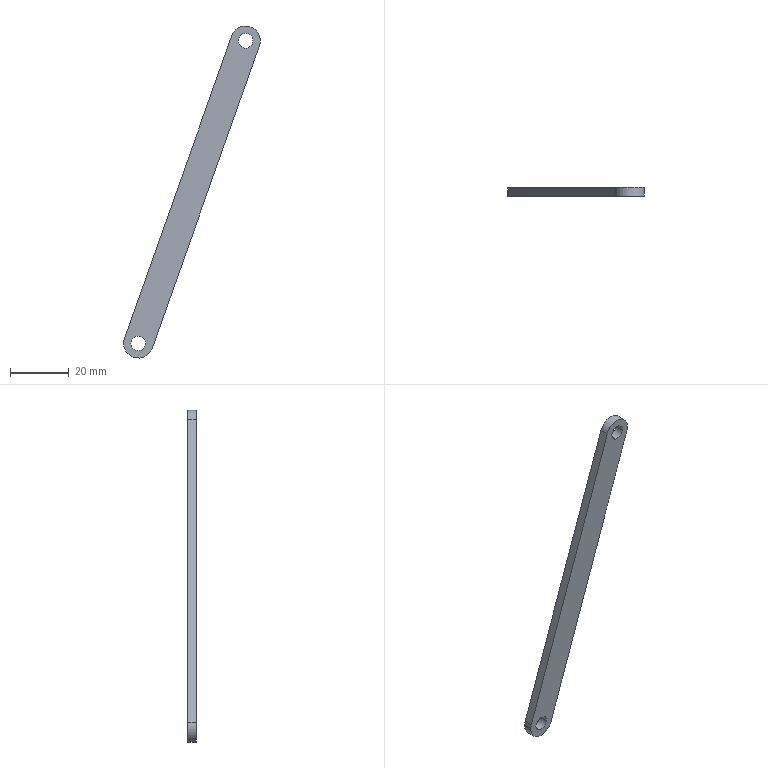Component | SolidWorks | WheelAssembly2-1_ConnectingRod2-1 | 1 solid | 11 faces | box 46.42 x 3 x 112.74 mm | volume 3388 mm3 | cylinder 7 | plane 4 | commonest cylinder face diameters 5 x4 10 x3
build123d program:
from build123d import *

# Parameters (mm, degrees)
SKETCH1_R           = 2.5
BOSS_EXTRUDE1_DEPTH = 3


with BuildPart() as part:
    # Sketch1 → Boss-Extrude1 (new body)
    with BuildSketch(Plane.XY):
        with BuildLine():
            Line((-54.5, 5), (54.5, 5))
            ThreePointArc((54.5, 5), (59.5, 0), (54.5, -5))
            Line((54.5, -5), (-54.5, -5))
            ThreePointArc((-54.5, -5), (-59.5, 0), (-54.5, 5))
        make_face()
        with Locations((-54.5, 0)):
            Circle(SKETCH1_R, mode=Mode.SUBTRACT)
        with Locations((54.5, 0)):
            Circle(SKETCH1_R, mode=Mode.SUBTRACT)
    extrude(amount=BOSS_EXTRUDE1_DEPTH)


solid = part.part

# Placed as in the assembly
solid = solid.moved(Location((-286.791, -33, -380.602), (-90, 0, -70.481)))
STEP:
#1=CARTESIAN_POINT('',(-10.607,-1.299,-13.055));
#2=VERTEX_POINT('',#1);
#3=CARTESIAN_POINT('',(-10.541,-1.299,-12.869));
#4=VERTEX_POINT('',#3);
#5=CARTESIAN_POINT('',(-10.574,-1.299,-12.962));
#6=DIRECTION('',(0.,-1.,0.));
#7=DIRECTION('',(0.3341,0.,0.9425));
#8=AXIS2_PLACEMENT_3D('',#5,#6,#7);
#9=CIRCLE('',#8,0.09843);
#10=EDGE_CURVE('',#2,#4,#9,.T.);
#11=ORIENTED_EDGE('',*,*,#10,.T.);
#12=CARTESIAN_POINT('',(-10.541,-1.181,-12.869));
#13=VERTEX_POINT('',#12);
#14=CARTESIAN_POINT('',(-10.541,-1.299,-12.869));
#15=DIRECTION('',(-0.,1.,-0.));
#16=VECTOR('',#15,39.37);
#17=LINE('',#14,#16);
#18=EDGE_CURVE('',#4,#13,#17,.T.);
#19=ORIENTED_EDGE('',*,*,#18,.T.);
#20=CARTESIAN_POINT('',(-10.607,-1.181,-13.055));
#21=VERTEX_POINT('',#20);
#22=CARTESIAN_POINT('',(-10.574,-1.181,-12.962));
#23=DIRECTION('',(0.,-1.,0.));
#24=DIRECTION('',(0.3341,0.,0.9425));
#25=AXIS2_PLACEMENT_3D('',#22,#23,#24);
#26=CIRCLE('',#25,0.09843);
#27=EDGE_CURVE('',#21,#13,#26,.T.);
#28=ORIENTED_EDGE('',*,*,#27,.F.);
#29=CARTESIAN_POINT('',(-10.607,-1.299,-13.055));
#30=DIRECTION('',(-0.,1.,-0.));
#31=VECTOR('',#30,39.37);
#32=LINE('',#29,#31);
#33=EDGE_CURVE('',#2,#21,#32,.T.);
#34=ORIENTED_EDGE('',*,*,#33,.F.);
#35=EDGE_LOOP('',(#11,#19,#28,#34));
#36=FACE_OUTER_BOUND('',#35,.T.);
#37=CARTESIAN_POINT('',(-10.574,-1.299,-12.962));
#38=DIRECTION('',(-0.,1.,-0.));
#39=DIRECTION('',(-0.3341,-0.,-0.9425));
#40=AXIS2_PLACEMENT_3D('',#37,#38,#39);
#41=CYLINDRICAL_SURFACE('',#40,0.09843);
#42=ADVANCED_FACE('',(#36),#41,.F.);
#43=CARTESIAN_POINT('',(-12.041,-1.299,-17.099));
#44=VERTEX_POINT('',#43);
#45=CARTESIAN_POINT('',(-11.975,-1.299,-16.914));
#46=VERTEX_POINT('',#45);
#47=CARTESIAN_POINT('',(-12.008,-1.299,-17.007));
#48=DIRECTION('',(0.,-1.,0.));
#49=DIRECTION('',(0.3341,0.,0.9425));
#50=AXIS2_PLACEMENT_3D('',#47,#48,#49);
#51=CIRCLE('',#50,0.09843);
#52=EDGE_CURVE('',#44,#46,#51,.T.);
#53=ORIENTED_EDGE('',*,*,#52,.T.);
#54=CARTESIAN_POINT('',(-11.975,-1.181,-16.914));
#55=VERTEX_POINT('',#54);
#56=CARTESIAN_POINT('',(-11.975,-1.299,-16.914));
#57=DIRECTION('',(-0.,1.,-0.));
#58=VECTOR('',#57,39.37);
#59=LINE('',#56,#58);
#60=EDGE_CURVE('',#46,#55,#59,.T.);
#61=ORIENTED_EDGE('',*,*,#60,.T.);
#62=CARTESIAN_POINT('',(-12.041,-1.181,-17.099));
#63=VERTEX_POINT('',#62);
#64=CARTESIAN_POINT('',(-12.008,-1.181,-17.007));
#65=DIRECTION('',(0.,-1.,0.));
#66=DIRECTION('',(0.3341,0.,0.9425));
#67=AXIS2_PLACEMENT_3D('',#64,#65,#66);
#68=CIRCLE('',#67,0.09843);
#69=EDGE_CURVE('',#63,#55,#68,.T.);
#70=ORIENTED_EDGE('',*,*,#69,.F.);
#71=CARTESIAN_POINT('',(-12.041,-1.299,-17.099));
#72=DIRECTION('',(-0.,1.,-0.));
#73=VECTOR('',#72,39.37);
#74=LINE('',#71,#73);
#75=EDGE_CURVE('',#44,#63,#74,.T.);
#76=ORIENTED_EDGE('',*,*,#75,.F.);
#77=EDGE_LOOP('',(#53,#61,#70,#76));
#78=FACE_OUTER_BOUND('',#77,.T.);
#79=CARTESIAN_POINT('',(-12.008,-1.299,-17.007));
#80=DIRECTION('',(-0.,1.,-0.));
#81=DIRECTION('',(-0.3341,-0.,-0.9425));
#82=AXIS2_PLACEMENT_3D('',#79,#80,#81);
#83=CYLINDRICAL_SURFACE('',#82,0.09843);
#84=ADVANCED_FACE('',(#78),#83,.F.);
#85=CARTESIAN_POINT('',(-12.074,-1.299,-17.192));
#86=VERTEX_POINT('',#85);
#87=CARTESIAN_POINT('',(-11.822,-1.299,-17.072));
#88=VERTEX_POINT('',#87);
#89=CARTESIAN_POINT('',(-12.008,-1.299,-17.007));
#90=DIRECTION('',(0.,-1.,0.));
#91=DIRECTION('',(0.3341,0.,0.9425));
#92=AXIS2_PLACEMENT_3D('',#89,#90,#91);
#93=CIRCLE('',#92,0.1969);
#94=EDGE_CURVE('',#86,#88,#93,.T.);
#95=ORIENTED_EDGE('',*,*,#94,.F.);
#96=CARTESIAN_POINT('',(-12.074,-1.181,-17.192));
#97=VERTEX_POINT('',#96);
#98=CARTESIAN_POINT('',(-12.074,-1.299,-17.192));
#99=DIRECTION('',(-0.,1.,-0.));
#100=VECTOR('',#99,39.37);
#101=LINE('',#98,#100);
#102=EDGE_CURVE('',#86,#97,#101,.T.);
#103=ORIENTED_EDGE('',*,*,#102,.T.);
#104=CARTESIAN_POINT('',(-11.822,-1.181,-17.072));
#105=VERTEX_POINT('',#104);
#106=CARTESIAN_POINT('',(-12.008,-1.181,-17.007));
#107=DIRECTION('',(0.,-1.,0.));
#108=DIRECTION('',(0.3341,0.,0.9425));
#109=AXIS2_PLACEMENT_3D('',#106,#107,#108);
#110=CIRCLE('',#109,0.1969);
#111=EDGE_CURVE('',#97,#105,#110,.T.);
#112=ORIENTED_EDGE('',*,*,#111,.T.);
#113=CARTESIAN_POINT('',(-11.822,-1.299,-17.072));
#114=DIRECTION('',(-0.,1.,-0.));
#115=VECTOR('',#114,39.37);
#116=LINE('',#113,#115);
#117=EDGE_CURVE('',#88,#105,#116,.T.);
#118=ORIENTED_EDGE('',*,*,#117,.F.);
#119=EDGE_LOOP('',(#95,#103,#112,#118));
#120=FACE_OUTER_BOUND('',#119,.T.);
#121=CARTESIAN_POINT('',(-12.008,-1.299,-17.007));
#122=DIRECTION('',(-0.,1.,-0.));
#123=DIRECTION('',(-0.3341,-0.,-0.9425));
#124=AXIS2_PLACEMENT_3D('',#121,#122,#123);
#125=CYLINDRICAL_SURFACE('',#124,0.1969);
#126=ADVANCED_FACE('',(#120),#125,.T.);
#127=ORIENTED_EDGE('',*,*,#52,.F.);
#128=CARTESIAN_POINT('',(-12.008,-1.299,-17.007));
#129=DIRECTION('',(0.,-1.,0.));
#130=DIRECTION('',(0.3341,0.,0.9425));
#131=AXIS2_PLACEMENT_3D('',#128,#129,#130);
#132=CIRCLE('',#131,0.09843);
#133=EDGE_CURVE('',#46,#44,#132,.T.);
#134=ORIENTED_EDGE('',*,*,#133,.F.);
#135=EDGE_LOOP('',(#127,#134));
#136=FACE_BOUND('',#135,.T.);
#137=CARTESIAN_POINT('',(-12.193,-1.299,-16.941));
#138=VERTEX_POINT('',#137);
#139=CARTESIAN_POINT('',(-12.008,-1.299,-17.007));
#140=DIRECTION('',(0.,-1.,0.));
#141=DIRECTION('',(0.3341,0.,0.9425));
#142=AXIS2_PLACEMENT_3D('',#139,#140,#141);
#143=CIRCLE('',#142,0.1969);
#144=EDGE_CURVE('',#138,#86,#143,.T.);
#145=ORIENTED_EDGE('',*,*,#144,.T.);
#146=ORIENTED_EDGE('',*,*,#94,.T.);
#147=CARTESIAN_POINT('',(-10.389,-1.299,-13.028));
#148=VERTEX_POINT('',#147);
#149=CARTESIAN_POINT('',(-11.822,-1.299,-17.072));
#150=DIRECTION('',(0.3341,0.,0.9425));
#151=VECTOR('',#150,39.37);
#152=LINE('',#149,#151);
#153=EDGE_CURVE('',#88,#148,#152,.T.);
#154=ORIENTED_EDGE('',*,*,#153,.T.);
#155=CARTESIAN_POINT('',(-10.76,-1.299,-12.896));
#156=VERTEX_POINT('',#155);
#157=CARTESIAN_POINT('',(-10.574,-1.299,-12.962));
#158=DIRECTION('',(0.,-1.,0.));
#159=DIRECTION('',(0.3341,0.,0.9425));
#160=AXIS2_PLACEMENT_3D('',#157,#158,#159);
#161=CIRCLE('',#160,0.1969);
#162=EDGE_CURVE('',#148,#156,#161,.T.);
#163=ORIENTED_EDGE('',*,*,#162,.T.);
#164=CARTESIAN_POINT('',(-12.193,-1.299,-16.941));
#165=DIRECTION('',(-0.3341,-0.,-0.9425));
#166=VECTOR('',#165,39.37);
#167=LINE('',#164,#166);
#168=EDGE_CURVE('',#156,#138,#167,.T.);
#169=ORIENTED_EDGE('',*,*,#168,.T.);
#170=EDGE_LOOP('',(#145,#146,#154,#163,#169));
#171=FACE_OUTER_BOUND('',#170,.T.);
#172=ORIENTED_EDGE('',*,*,#10,.F.);
#173=CARTESIAN_POINT('',(-10.574,-1.299,-12.962));
#174=DIRECTION('',(0.,-1.,0.));
#175=DIRECTION('',(0.3341,0.,0.9425));
#176=AXIS2_PLACEMENT_3D('',#173,#174,#175);
#177=CIRCLE('',#176,0.09843);
#178=EDGE_CURVE('',#4,#2,#177,.T.);
#179=ORIENTED_EDGE('',*,*,#178,.F.);
#180=EDGE_LOOP('',(#172,#179));
#181=FACE_BOUND('',#180,.T.);
#182=CARTESIAN_POINT('',(-12.008,-1.299,-17.007));
#183=DIRECTION('',(0.,-1.,0.));
#184=DIRECTION('',(0.3341,0.,0.9425));
#185=AXIS2_PLACEMENT_3D('',#182,#183,#184);
#186=PLANE('',#185);
#187=ADVANCED_FACE('',(#136,#171,#181),#186,.T.);
#188=CARTESIAN_POINT('',(-12.193,-1.181,-16.941));
#189=VERTEX_POINT('',#188);
#190=CARTESIAN_POINT('',(-12.008,-1.181,-17.007));
#191=DIRECTION('',(0.,-1.,0.));
#192=DIRECTION('',(0.3341,0.,0.9425));
#193=AXIS2_PLACEMENT_3D('',#190,#191,#192);
#194=CIRCLE('',#193,0.1969);
#195=EDGE_CURVE('',#189,#97,#194,.T.);
#196=ORIENTED_EDGE('',*,*,#195,.F.);
#197=CARTESIAN_POINT('',(-10.76,-1.181,-12.896));
#198=VERTEX_POINT('',#197);
#199=CARTESIAN_POINT('',(-12.193,-1.181,-16.941));
#200=DIRECTION('',(-0.3341,-0.,-0.9425));
#201=VECTOR('',#200,39.37);
#202=LINE('',#199,#201);
#203=EDGE_CURVE('',#198,#189,#202,.T.);
#204=ORIENTED_EDGE('',*,*,#203,.F.);
#205=CARTESIAN_POINT('',(-10.389,-1.181,-13.028));
#206=VERTEX_POINT('',#205);
#207=CARTESIAN_POINT('',(-10.574,-1.181,-12.962));
#208=DIRECTION('',(0.,-1.,0.));
#209=DIRECTION('',(0.3341,0.,0.9425));
#210=AXIS2_PLACEMENT_3D('',#207,#208,#209);
#211=CIRCLE('',#210,0.1969);
#212=EDGE_CURVE('',#206,#198,#211,.T.);
#213=ORIENTED_EDGE('',*,*,#212,.F.);
#214=CARTESIAN_POINT('',(-11.822,-1.181,-17.072));
#215=DIRECTION('',(0.3341,0.,0.9425));
#216=VECTOR('',#215,39.37);
#217=LINE('',#214,#216);
#218=EDGE_CURVE('',#105,#206,#217,.T.);
#219=ORIENTED_EDGE('',*,*,#218,.F.);
#220=ORIENTED_EDGE('',*,*,#111,.F.);
#221=EDGE_LOOP('',(#196,#204,#213,#219,#220));
#222=FACE_OUTER_BOUND('',#221,.T.);
#223=ORIENTED_EDGE('',*,*,#69,.T.);
#224=CARTESIAN_POINT('',(-12.008,-1.181,-17.007));
#225=DIRECTION('',(0.,-1.,0.));
#226=DIRECTION('',(0.3341,0.,0.9425));
#227=AXIS2_PLACEMENT_3D('',#224,#225,#226);
#228=CIRCLE('',#227,0.09843);
#229=EDGE_CURVE('',#55,#63,#228,.T.);
#230=ORIENTED_EDGE('',*,*,#229,.T.);
#231=EDGE_LOOP('',(#223,#230));
#232=FACE_BOUND('',#231,.T.);
#233=ORIENTED_EDGE('',*,*,#27,.T.);
#234=CARTESIAN_POINT('',(-10.574,-1.181,-12.962));
#235=DIRECTION('',(0.,-1.,0.));
#236=DIRECTION('',(0.3341,0.,0.9425));
#237=AXIS2_PLACEMENT_3D('',#234,#235,#236);
#238=CIRCLE('',#237,0.09843);
#239=EDGE_CURVE('',#13,#21,#238,.T.);
#240=ORIENTED_EDGE('',*,*,#239,.T.);
#241=EDGE_LOOP('',(#233,#240));
#242=FACE_BOUND('',#241,.T.);
#243=CARTESIAN_POINT('',(-12.008,-1.181,-17.007));
#244=DIRECTION('',(0.,-1.,0.));
#245=DIRECTION('',(0.3341,0.,0.9425));
#246=AXIS2_PLACEMENT_3D('',#243,#244,#245);
#247=PLANE('',#246);
#248=ADVANCED_FACE('',(#222,#232,#242),#247,.F.);
#249=ORIENTED_EDGE('',*,*,#102,.F.);
#250=ORIENTED_EDGE('',*,*,#144,.F.);
#251=CARTESIAN_POINT('',(-12.193,-1.299,-16.941));
#252=DIRECTION('',(-0.,1.,-0.));
#253=VECTOR('',#252,39.37);
#254=LINE('',#251,#253);
#255=EDGE_CURVE('',#138,#189,#254,.T.);
#256=ORIENTED_EDGE('',*,*,#255,.T.);
#257=ORIENTED_EDGE('',*,*,#195,.T.);
#258=EDGE_LOOP('',(#249,#250,#256,#257));
#259=FACE_OUTER_BOUND('',#258,.T.);
#260=CARTESIAN_POINT('',(-12.008,-1.299,-17.007));
#261=DIRECTION('',(-0.,1.,-0.));
#262=DIRECTION('',(-0.3341,-0.,-0.9425));
#263=AXIS2_PLACEMENT_3D('',#260,#261,#262);
#264=CYLINDRICAL_SURFACE('',#263,0.1969);
#265=ADVANCED_FACE('',(#259),#264,.T.);
#266=ORIENTED_EDGE('',*,*,#218,.T.);
#267=CARTESIAN_POINT('',(-10.389,-1.299,-13.028));
#268=DIRECTION('',(-0.,1.,-0.));
#269=VECTOR('',#268,39.37);
#270=LINE('',#267,#269);
#271=EDGE_CURVE('',#148,#206,#270,.T.);
#272=ORIENTED_EDGE('',*,*,#271,.F.);
#273=ORIENTED_EDGE('',*,*,#153,.F.);
#274=ORIENTED_EDGE('',*,*,#117,.T.);
#275=EDGE_LOOP('',(#266,#272,#273,#274));
#276=FACE_OUTER_BOUND('',#275,.T.);
#277=CARTESIAN_POINT('',(-11.822,-1.299,-17.072));
#278=DIRECTION('',(-0.9425,-0.,0.3341));
#279=DIRECTION('',(0.,-1.,0.));
#280=AXIS2_PLACEMENT_3D('',#277,#278,#279);
#281=PLANE('',#280);
#282=ADVANCED_FACE('',(#276),#281,.F.);
#283=ORIENTED_EDGE('',*,*,#212,.T.);
#284=CARTESIAN_POINT('',(-10.76,-1.299,-12.896));
#285=DIRECTION('',(-0.,1.,-0.));
#286=VECTOR('',#285,39.37);
#287=LINE('',#284,#286);
#288=EDGE_CURVE('',#156,#198,#287,.T.);
#289=ORIENTED_EDGE('',*,*,#288,.F.);
#290=ORIENTED_EDGE('',*,*,#162,.F.);
#291=ORIENTED_EDGE('',*,*,#271,.T.);
#292=EDGE_LOOP('',(#283,#289,#290,#291));
#293=FACE_OUTER_BOUND('',#292,.T.);
#294=CARTESIAN_POINT('',(-10.574,-1.299,-12.962));
#295=DIRECTION('',(-0.,1.,-0.));
#296=DIRECTION('',(-0.3341,-0.,-0.9425));
#297=AXIS2_PLACEMENT_3D('',#294,#295,#296);
#298=CYLINDRICAL_SURFACE('',#297,0.1969);
#299=ADVANCED_FACE('',(#293),#298,.T.);
#300=ORIENTED_EDGE('',*,*,#203,.T.);
#301=ORIENTED_EDGE('',*,*,#255,.F.);
#302=ORIENTED_EDGE('',*,*,#168,.F.);
#303=ORIENTED_EDGE('',*,*,#288,.T.);
#304=EDGE_LOOP('',(#300,#301,#302,#303));
#305=FACE_OUTER_BOUND('',#304,.T.);
#306=CARTESIAN_POINT('',(-12.193,-1.299,-16.941));
#307=DIRECTION('',(0.9425,0.,-0.3341));
#308=DIRECTION('',(0.3341,0.,0.9425));
#309=AXIS2_PLACEMENT_3D('',#306,#307,#308);
#310=PLANE('',#309);
#311=ADVANCED_FACE('',(#305),#310,.F.);
#312=ORIENTED_EDGE('',*,*,#60,.F.);
#313=ORIENTED_EDGE('',*,*,#133,.T.);
#314=ORIENTED_EDGE('',*,*,#75,.T.);
#315=ORIENTED_EDGE('',*,*,#229,.F.);
#316=EDGE_LOOP('',(#312,#313,#314,#315));
#317=FACE_OUTER_BOUND('',#316,.T.);
#318=CARTESIAN_POINT('',(-12.008,-1.299,-17.007));
#319=DIRECTION('',(-0.,1.,-0.));
#320=DIRECTION('',(-0.3341,-0.,-0.9425));
#321=AXIS2_PLACEMENT_3D('',#318,#319,#320);
#322=CYLINDRICAL_SURFACE('',#321,0.09843);
#323=ADVANCED_FACE('',(#317),#322,.F.);
#324=ORIENTED_EDGE('',*,*,#18,.F.);
#325=ORIENTED_EDGE('',*,*,#178,.T.);
#326=ORIENTED_EDGE('',*,*,#33,.T.);
#327=ORIENTED_EDGE('',*,*,#239,.F.);
#328=EDGE_LOOP('',(#324,#325,#326,#327));
#329=FACE_OUTER_BOUND('',#328,.T.);
#330=CARTESIAN_POINT('',(-10.574,-1.299,-12.962));
#331=DIRECTION('',(-0.,1.,-0.));
#332=DIRECTION('',(-0.3341,-0.,-0.9425));
#333=AXIS2_PLACEMENT_3D('',#330,#331,#332);
#334=CYLINDRICAL_SURFACE('',#333,0.09843);
#335=ADVANCED_FACE('',(#329),#334,.F.);
#336=CLOSED_SHELL('',(#42,#84,#126,#187,#248,#265,#282,#299,#311,#323,#335));
#337=MANIFOLD_SOLID_BREP('',#336);
#338=CARTESIAN_POINT('',(0.,0.,0.));
#339=DIRECTION('',(0.,0.,1.));
#340=DIRECTION('',(1.,0.,0.));
#341=AXIS2_PLACEMENT_3D('',#338,#339,#340);
#342=(LENGTH_UNIT()NAMED_UNIT(*)SI_UNIT($,.METRE.));
#343=LENGTH_MEASURE_WITH_UNIT(LENGTH_MEASURE(0.0254),#342);
#344=DIMENSIONAL_EXPONENTS(1.,0.,0.,0.,0.,0.,0.);
#345=(CONVERSION_BASED_UNIT('',#343)LENGTH_UNIT()NAMED_UNIT(#344));
#346=UNCERTAINTY_MEASURE_WITH_UNIT(LENGTH_MEASURE(0.00001),#345,'','');
#347=(NAMED_UNIT(*)PLANE_ANGLE_UNIT()SI_UNIT($,.RADIAN.));
#348=(NAMED_UNIT(*)SI_UNIT($,.STERADIAN.)SOLID_ANGLE_UNIT());
#349=(GEOMETRIC_REPRESENTATION_CONTEXT(3)GLOBAL_UNCERTAINTY_ASSIGNED_CONTEXT((#346))GLOBAL_UNIT_ASSIGNED_CONTEXT((#345,#347,#348))REPRESENTATION_CONTEXT('',''));
#350=ADVANCED_BREP_SHAPE_REPRESENTATION('',(#337,#341),#349);
#351=COLOUR_RGB('',0.7922,0.8196,0.9333);
#352=FILL_AREA_STYLE_COLOUR('',#351);
#353=FILL_AREA_STYLE('',(#352));
#354=SURFACE_STYLE_FILL_AREA(#353);
#355=SURFACE_SIDE_STYLE('',(#354));
#356=SURFACE_STYLE_USAGE(.BOTH.,#355);
#357=PRESENTATION_STYLE_ASSIGNMENT((#356));
#358=STYLED_ITEM('',(#357),#337);
#359=PRESENTATION_LAYER_ASSIGNMENT('','',(#358));
#360=(LENGTH_UNIT()NAMED_UNIT(*)SI_UNIT($,.METRE.));
#361=LENGTH_MEASURE_WITH_UNIT(LENGTH_MEASURE(0.0254),#360);
#362=DIMENSIONAL_EXPONENTS(1.,0.,0.,0.,0.,0.,0.);
#363=(CONVERSION_BASED_UNIT('',#361)LENGTH_UNIT()NAMED_UNIT(#362));
#364=UNCERTAINTY_MEASURE_WITH_UNIT(LENGTH_MEASURE(0.00001),#363,'','');
#365=(NAMED_UNIT(*)PLANE_ANGLE_UNIT()SI_UNIT($,.RADIAN.));
#366=(NAMED_UNIT(*)SI_UNIT($,.STERADIAN.)SOLID_ANGLE_UNIT());
#367=(GEOMETRIC_REPRESENTATION_CONTEXT(3)GLOBAL_UNCERTAINTY_ASSIGNED_CONTEXT((#364))GLOBAL_UNIT_ASSIGNED_CONTEXT((#363,#365,#366))REPRESENTATION_CONTEXT('',''));
#368=MECHANICAL_DESIGN_GEOMETRIC_PRESENTATION_REPRESENTATION('',(#358),#367);